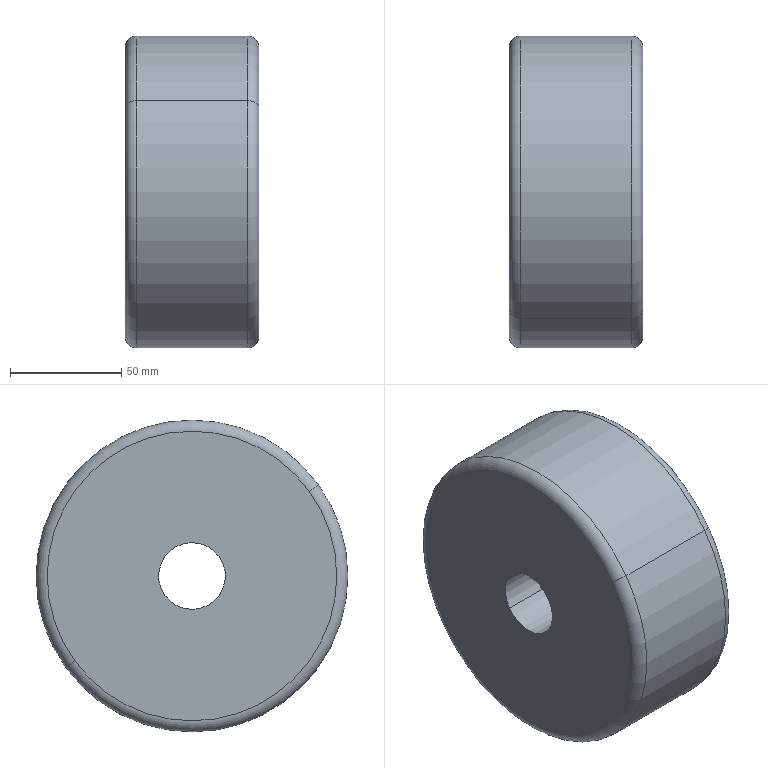Component | SolidWorks | TrashCanWheel-3 | 1 solid | 10 faces | box 60 x 140 x 140 mm | volume 876573 mm3 | torus 4 | cylinder 4 | plane 2 | commonest cylinder face diameters 30 x2 140 x2
build123d program:
from build123d import *

# Parameters (mm, degrees)
SKETCH1_R           = 70
SKETCH1_R_2         = 15
BOSS_EXTRUDE1_DEPTH = 60
FILLET1_R           = 5


with BuildPart() as part:
    # Sketch1 → Boss-Extrude1 (new body)
    with BuildSketch(Plane.XY):
        Circle(SKETCH1_R)
        Circle(SKETCH1_R_2, mode=Mode.SUBTRACT)
    extrude(amount=BOSS_EXTRUDE1_DEPTH)

    # Fillet1
    fillet1_edges = [part.edges().sort_by_distance(p)[0] for p in [
        (-70, 0, 0),
        (-70, 0, 60),
    ]]
    fillet(fillet1_edges, radius=FILLET1_R)


solid = part.part

# Placed as in the assembly
solid = solid.moved(Location((-414.371, -1323.331, 8.161), (0, 90, 0)))
STEP:
#1=CARTESIAN_POINT('',(-16.117,-49.866,-1.293));
#2=VERTEX_POINT('',#1);
#3=CARTESIAN_POINT('',(-16.117,-54.333,1.935));
#4=VERTEX_POINT('',#3);
#5=CARTESIAN_POINT('',(-16.117,-52.1,0.3213));
#6=DIRECTION('',(1.,0.,-0.));
#7=DIRECTION('',(0.,-0.8105,0.5857));
#8=AXIS2_PLACEMENT_3D('',#5,#6,#7);
#9=CIRCLE('',#8,2.756);
#10=EDGE_CURVE('',#2,#4,#9,.T.);
#11=ORIENTED_EDGE('',*,*,#10,.F.);
#12=CARTESIAN_POINT('',(-16.314,-50.025,-1.177));
#13=VERTEX_POINT('',#12);
#14=CARTESIAN_POINT('',(-16.117,-50.025,-1.177));
#15=DIRECTION('',(0.,0.5857,0.8105));
#16=DIRECTION('',(0.,-0.8105,0.5857));
#17=AXIS2_PLACEMENT_3D('',#14,#15,#16);
#18=CIRCLE('',#17,0.1969);
#19=EDGE_CURVE('',#2,#13,#18,.T.);
#20=ORIENTED_EDGE('',*,*,#19,.T.);
#21=CARTESIAN_POINT('',(-16.314,-54.174,1.82));
#22=VERTEX_POINT('',#21);
#23=CARTESIAN_POINT('',(-16.314,-52.1,0.3213));
#24=DIRECTION('',(-1.,-0.,0.));
#25=DIRECTION('',(0.,-0.8105,0.5857));
#26=AXIS2_PLACEMENT_3D('',#23,#24,#25);
#27=CIRCLE('',#26,2.559);
#28=EDGE_CURVE('',#22,#13,#27,.T.);
#29=ORIENTED_EDGE('',*,*,#28,.F.);
#30=CARTESIAN_POINT('',(-16.117,-54.174,1.82));
#31=DIRECTION('',(-0.,-0.5857,-0.8105));
#32=DIRECTION('',(0.,0.8105,-0.5857));
#33=AXIS2_PLACEMENT_3D('',#30,#31,#32);
#34=CIRCLE('',#33,0.1969);
#35=EDGE_CURVE('',#4,#22,#34,.T.);
#36=ORIENTED_EDGE('',*,*,#35,.F.);
#37=EDGE_LOOP('',(#11,#20,#29,#36));
#38=FACE_OUTER_BOUND('',#37,.T.);
#39=CARTESIAN_POINT('',(-16.117,-52.1,0.3213));
#40=DIRECTION('',(-1.,-0.,0.));
#41=DIRECTION('',(0.,-0.8105,0.5857));
#42=AXIS2_PLACEMENT_3D('',#39,#40,#41);
#43=TOROIDAL_SURFACE('',#42,2.559,0.1969);
#44=ADVANCED_FACE('',(#38),#43,.T.);
#45=CARTESIAN_POINT('',(-13.952,-50.025,-1.177));
#46=VERTEX_POINT('',#45);
#47=CARTESIAN_POINT('',(-13.952,-54.174,1.82));
#48=VERTEX_POINT('',#47);
#49=CARTESIAN_POINT('',(-13.952,-52.1,0.3213));
#50=DIRECTION('',(1.,0.,-0.));
#51=DIRECTION('',(0.,-0.8105,0.5857));
#52=AXIS2_PLACEMENT_3D('',#49,#50,#51);
#53=CIRCLE('',#52,2.559);
#54=EDGE_CURVE('',#46,#48,#53,.T.);
#55=ORIENTED_EDGE('',*,*,#54,.F.);
#56=CARTESIAN_POINT('',(-14.148,-49.866,-1.293));
#57=VERTEX_POINT('',#56);
#58=CARTESIAN_POINT('',(-14.148,-50.025,-1.177));
#59=DIRECTION('',(0.,0.5857,0.8105));
#60=DIRECTION('',(0.,-0.8105,0.5857));
#61=AXIS2_PLACEMENT_3D('',#58,#59,#60);
#62=CIRCLE('',#61,0.1969);
#63=EDGE_CURVE('',#46,#57,#62,.T.);
#64=ORIENTED_EDGE('',*,*,#63,.T.);
#65=CARTESIAN_POINT('',(-14.148,-54.333,1.935));
#66=VERTEX_POINT('',#65);
#67=CARTESIAN_POINT('',(-14.148,-52.1,0.3213));
#68=DIRECTION('',(-1.,-0.,0.));
#69=DIRECTION('',(0.,-0.8105,0.5857));
#70=AXIS2_PLACEMENT_3D('',#67,#68,#69);
#71=CIRCLE('',#70,2.756);
#72=EDGE_CURVE('',#66,#57,#71,.T.);
#73=ORIENTED_EDGE('',*,*,#72,.F.);
#74=CARTESIAN_POINT('',(-14.148,-54.174,1.82));
#75=DIRECTION('',(-0.,-0.5857,-0.8105));
#76=DIRECTION('',(0.,0.8105,-0.5857));
#77=AXIS2_PLACEMENT_3D('',#74,#75,#76);
#78=CIRCLE('',#77,0.1969);
#79=EDGE_CURVE('',#48,#66,#78,.T.);
#80=ORIENTED_EDGE('',*,*,#79,.F.);
#81=EDGE_LOOP('',(#55,#64,#73,#80));
#82=FACE_OUTER_BOUND('',#81,.T.);
#83=CARTESIAN_POINT('',(-14.148,-52.1,0.3213));
#84=DIRECTION('',(-1.,-0.,0.));
#85=DIRECTION('',(0.,-0.8105,0.5857));
#86=AXIS2_PLACEMENT_3D('',#83,#84,#85);
#87=TOROIDAL_SURFACE('',#86,2.559,0.1969);
#88=ADVANCED_FACE('',(#82),#87,.T.);
#89=CARTESIAN_POINT('',(-16.314,-51.621,-0.02458));
#90=VERTEX_POINT('',#89);
#91=CARTESIAN_POINT('',(-16.314,-52.578,0.6672));
#92=VERTEX_POINT('',#91);
#93=CARTESIAN_POINT('',(-16.314,-52.1,0.3213));
#94=DIRECTION('',(-1.,-0.,0.));
#95=DIRECTION('',(0.,-0.8105,0.5857));
#96=AXIS2_PLACEMENT_3D('',#93,#94,#95);
#97=CIRCLE('',#96,0.5906);
#98=EDGE_CURVE('',#90,#92,#97,.T.);
#99=ORIENTED_EDGE('',*,*,#98,.T.);
#100=CARTESIAN_POINT('',(-13.952,-52.578,0.6672));
#101=VERTEX_POINT('',#100);
#102=CARTESIAN_POINT('',(-16.314,-52.578,0.6672));
#103=DIRECTION('',(1.,0.,-0.));
#104=VECTOR('',#103,39.37);
#105=LINE('',#102,#104);
#106=EDGE_CURVE('',#92,#101,#105,.T.);
#107=ORIENTED_EDGE('',*,*,#106,.T.);
#108=CARTESIAN_POINT('',(-13.952,-51.621,-0.02458));
#109=VERTEX_POINT('',#108);
#110=CARTESIAN_POINT('',(-13.952,-52.1,0.3213));
#111=DIRECTION('',(-1.,-0.,0.));
#112=DIRECTION('',(0.,-0.8105,0.5857));
#113=AXIS2_PLACEMENT_3D('',#110,#111,#112);
#114=CIRCLE('',#113,0.5906);
#115=EDGE_CURVE('',#109,#101,#114,.T.);
#116=ORIENTED_EDGE('',*,*,#115,.F.);
#117=CARTESIAN_POINT('',(-16.314,-51.621,-0.02458));
#118=DIRECTION('',(1.,0.,-0.));
#119=VECTOR('',#118,39.37);
#120=LINE('',#117,#119);
#121=EDGE_CURVE('',#90,#109,#120,.T.);
#122=ORIENTED_EDGE('',*,*,#121,.F.);
#123=EDGE_LOOP('',(#99,#107,#116,#122));
#124=FACE_OUTER_BOUND('',#123,.T.);
#125=CARTESIAN_POINT('',(-16.314,-52.1,0.3213));
#126=DIRECTION('',(1.,0.,-0.));
#127=DIRECTION('',(0.,0.8105,-0.5857));
#128=AXIS2_PLACEMENT_3D('',#125,#126,#127);
#129=CYLINDRICAL_SURFACE('',#128,0.5906);
#130=ADVANCED_FACE('',(#124),#129,.F.);
#131=ORIENTED_EDGE('',*,*,#10,.T.);
#132=CARTESIAN_POINT('',(-16.314,-54.333,1.935));
#133=DIRECTION('',(1.,0.,-0.));
#134=VECTOR('',#133,39.37);
#135=LINE('',#132,#134);
#136=EDGE_CURVE('',#4,#66,#135,.T.);
#137=ORIENTED_EDGE('',*,*,#136,.T.);
#138=ORIENTED_EDGE('',*,*,#72,.T.);
#139=CARTESIAN_POINT('',(-16.314,-49.866,-1.293));
#140=DIRECTION('',(1.,0.,-0.));
#141=VECTOR('',#140,39.37);
#142=LINE('',#139,#141);
#143=EDGE_CURVE('',#2,#57,#142,.T.);
#144=ORIENTED_EDGE('',*,*,#143,.F.);
#145=EDGE_LOOP('',(#131,#137,#138,#144));
#146=FACE_OUTER_BOUND('',#145,.T.);
#147=CARTESIAN_POINT('',(-16.314,-52.1,0.3213));
#148=DIRECTION('',(1.,0.,-0.));
#149=DIRECTION('',(0.,0.8105,-0.5857));
#150=AXIS2_PLACEMENT_3D('',#147,#148,#149);
#151=CYLINDRICAL_SURFACE('',#150,2.756);
#152=ADVANCED_FACE('',(#146),#151,.T.);
#153=ORIENTED_EDGE('',*,*,#28,.T.);
#154=CARTESIAN_POINT('',(-16.314,-52.1,0.3213));
#155=DIRECTION('',(-1.,-0.,0.));
#156=DIRECTION('',(0.,-0.8105,0.5857));
#157=AXIS2_PLACEMENT_3D('',#154,#155,#156);
#158=CIRCLE('',#157,2.559);
#159=EDGE_CURVE('',#13,#22,#158,.T.);
#160=ORIENTED_EDGE('',*,*,#159,.T.);
#161=EDGE_LOOP('',(#153,#160));
#162=FACE_OUTER_BOUND('',#161,.T.);
#163=ORIENTED_EDGE('',*,*,#98,.F.);
#164=CARTESIAN_POINT('',(-16.314,-52.1,0.3213));
#165=DIRECTION('',(-1.,-0.,0.));
#166=DIRECTION('',(0.,-0.8105,0.5857));
#167=AXIS2_PLACEMENT_3D('',#164,#165,#166);
#168=CIRCLE('',#167,0.5906);
#169=EDGE_CURVE('',#92,#90,#168,.T.);
#170=ORIENTED_EDGE('',*,*,#169,.F.);
#171=EDGE_LOOP('',(#163,#170));
#172=FACE_BOUND('',#171,.T.);
#173=CARTESIAN_POINT('',(-16.314,-52.1,0.3213));
#174=DIRECTION('',(-1.,-0.,0.));
#175=DIRECTION('',(0.,-0.8105,0.5857));
#176=AXIS2_PLACEMENT_3D('',#173,#174,#175);
#177=PLANE('',#176);
#178=ADVANCED_FACE('',(#162,#172),#177,.T.);
#179=CARTESIAN_POINT('',(-13.952,-52.1,0.3213));
#180=DIRECTION('',(1.,0.,-0.));
#181=DIRECTION('',(0.,-0.8105,0.5857));
#182=AXIS2_PLACEMENT_3D('',#179,#180,#181);
#183=CIRCLE('',#182,2.559);
#184=EDGE_CURVE('',#48,#46,#183,.T.);
#185=ORIENTED_EDGE('',*,*,#184,.T.);
#186=ORIENTED_EDGE('',*,*,#54,.T.);
#187=EDGE_LOOP('',(#185,#186));
#188=FACE_OUTER_BOUND('',#187,.T.);
#189=ORIENTED_EDGE('',*,*,#115,.T.);
#190=CARTESIAN_POINT('',(-13.952,-52.1,0.3213));
#191=DIRECTION('',(-1.,-0.,0.));
#192=DIRECTION('',(0.,-0.8105,0.5857));
#193=AXIS2_PLACEMENT_3D('',#190,#191,#192);
#194=CIRCLE('',#193,0.5906);
#195=EDGE_CURVE('',#101,#109,#194,.T.);
#196=ORIENTED_EDGE('',*,*,#195,.T.);
#197=EDGE_LOOP('',(#189,#196));
#198=FACE_BOUND('',#197,.T.);
#199=CARTESIAN_POINT('',(-13.952,-52.1,0.3213));
#200=DIRECTION('',(-1.,-0.,0.));
#201=DIRECTION('',(0.,-0.8105,0.5857));
#202=AXIS2_PLACEMENT_3D('',#199,#200,#201);
#203=PLANE('',#202);
#204=ADVANCED_FACE('',(#188,#198),#203,.F.);
#205=ORIENTED_EDGE('',*,*,#136,.F.);
#206=CARTESIAN_POINT('',(-16.117,-52.1,0.3213));
#207=DIRECTION('',(1.,0.,-0.));
#208=DIRECTION('',(0.,-0.8105,0.5857));
#209=AXIS2_PLACEMENT_3D('',#206,#207,#208);
#210=CIRCLE('',#209,2.756);
#211=EDGE_CURVE('',#4,#2,#210,.T.);
#212=ORIENTED_EDGE('',*,*,#211,.T.);
#213=ORIENTED_EDGE('',*,*,#143,.T.);
#214=CARTESIAN_POINT('',(-14.148,-52.1,0.3213));
#215=DIRECTION('',(-1.,-0.,0.));
#216=DIRECTION('',(0.,-0.8105,0.5857));
#217=AXIS2_PLACEMENT_3D('',#214,#215,#216);
#218=CIRCLE('',#217,2.756);
#219=EDGE_CURVE('',#57,#66,#218,.T.);
#220=ORIENTED_EDGE('',*,*,#219,.T.);
#221=EDGE_LOOP('',(#205,#212,#213,#220));
#222=FACE_OUTER_BOUND('',#221,.T.);
#223=CARTESIAN_POINT('',(-16.314,-52.1,0.3213));
#224=DIRECTION('',(1.,0.,-0.));
#225=DIRECTION('',(0.,0.8105,-0.5857));
#226=AXIS2_PLACEMENT_3D('',#223,#224,#225);
#227=CYLINDRICAL_SURFACE('',#226,2.756);
#228=ADVANCED_FACE('',(#222),#227,.T.);
#229=ORIENTED_EDGE('',*,*,#106,.F.);
#230=ORIENTED_EDGE('',*,*,#169,.T.);
#231=ORIENTED_EDGE('',*,*,#121,.T.);
#232=ORIENTED_EDGE('',*,*,#195,.F.);
#233=EDGE_LOOP('',(#229,#230,#231,#232));
#234=FACE_OUTER_BOUND('',#233,.T.);
#235=CARTESIAN_POINT('',(-16.314,-52.1,0.3213));
#236=DIRECTION('',(1.,0.,-0.));
#237=DIRECTION('',(0.,0.8105,-0.5857));
#238=AXIS2_PLACEMENT_3D('',#235,#236,#237);
#239=CYLINDRICAL_SURFACE('',#238,0.5906);
#240=ADVANCED_FACE('',(#234),#239,.F.);
#241=ORIENTED_EDGE('',*,*,#63,.F.);
#242=ORIENTED_EDGE('',*,*,#184,.F.);
#243=ORIENTED_EDGE('',*,*,#79,.T.);
#244=ORIENTED_EDGE('',*,*,#219,.F.);
#245=EDGE_LOOP('',(#241,#242,#243,#244));
#246=FACE_OUTER_BOUND('',#245,.T.);
#247=CARTESIAN_POINT('',(-14.148,-52.1,0.3213));
#248=DIRECTION('',(-1.,-0.,0.));
#249=DIRECTION('',(0.,-0.8105,0.5857));
#250=AXIS2_PLACEMENT_3D('',#247,#248,#249);
#251=TOROIDAL_SURFACE('',#250,2.559,0.1969);
#252=ADVANCED_FACE('',(#246),#251,.T.);
#253=ORIENTED_EDGE('',*,*,#19,.F.);
#254=ORIENTED_EDGE('',*,*,#211,.F.);
#255=ORIENTED_EDGE('',*,*,#35,.T.);
#256=ORIENTED_EDGE('',*,*,#159,.F.);
#257=EDGE_LOOP('',(#253,#254,#255,#256));
#258=FACE_OUTER_BOUND('',#257,.T.);
#259=CARTESIAN_POINT('',(-16.117,-52.1,0.3213));
#260=DIRECTION('',(-1.,-0.,0.));
#261=DIRECTION('',(0.,-0.8105,0.5857));
#262=AXIS2_PLACEMENT_3D('',#259,#260,#261);
#263=TOROIDAL_SURFACE('',#262,2.559,0.1969);
#264=ADVANCED_FACE('',(#258),#263,.T.);
#265=CLOSED_SHELL('',(#44,#88,#130,#152,#178,#204,#228,#240,#252,#264));
#266=MANIFOLD_SOLID_BREP('',#265);
#267=CARTESIAN_POINT('',(0.,0.,0.));
#268=DIRECTION('',(0.,0.,1.));
#269=DIRECTION('',(1.,0.,0.));
#270=AXIS2_PLACEMENT_3D('',#267,#268,#269);
#271=(LENGTH_UNIT()NAMED_UNIT(*)SI_UNIT($,.METRE.));
#272=LENGTH_MEASURE_WITH_UNIT(LENGTH_MEASURE(0.0254),#271);
#273=DIMENSIONAL_EXPONENTS(1.,0.,0.,0.,0.,0.,0.);
#274=(CONVERSION_BASED_UNIT('',#272)LENGTH_UNIT()NAMED_UNIT(#273));
#275=UNCERTAINTY_MEASURE_WITH_UNIT(LENGTH_MEASURE(0.00001),#274,'','');
#276=(NAMED_UNIT(*)PLANE_ANGLE_UNIT()SI_UNIT($,.RADIAN.));
#277=(NAMED_UNIT(*)SI_UNIT($,.STERADIAN.)SOLID_ANGLE_UNIT());
#278=(GEOMETRIC_REPRESENTATION_CONTEXT(3)GLOBAL_UNCERTAINTY_ASSIGNED_CONTEXT((#275))GLOBAL_UNIT_ASSIGNED_CONTEXT((#274,#276,#277))REPRESENTATION_CONTEXT('',''));
#279=ADVANCED_BREP_SHAPE_REPRESENTATION('',(#266,#270),#278);
#280=COLOUR_RGB('',0.7922,0.8196,0.9333);
#281=FILL_AREA_STYLE_COLOUR('',#280);
#282=FILL_AREA_STYLE('',(#281));
#283=SURFACE_STYLE_FILL_AREA(#282);
#284=SURFACE_SIDE_STYLE('',(#283));
#285=SURFACE_STYLE_USAGE(.BOTH.,#284);
#286=PRESENTATION_STYLE_ASSIGNMENT((#285));
#287=STYLED_ITEM('',(#286),#266);
#288=(LENGTH_UNIT()NAMED_UNIT(*)SI_UNIT($,.METRE.));
#289=LENGTH_MEASURE_WITH_UNIT(LENGTH_MEASURE(0.0254),#288);
#290=DIMENSIONAL_EXPONENTS(1.,0.,0.,0.,0.,0.,0.);
#291=(CONVERSION_BASED_UNIT('',#289)LENGTH_UNIT()NAMED_UNIT(#290));
#292=UNCERTAINTY_MEASURE_WITH_UNIT(LENGTH_MEASURE(0.00001),#291,'','');
#293=(NAMED_UNIT(*)PLANE_ANGLE_UNIT()SI_UNIT($,.RADIAN.));
#294=(NAMED_UNIT(*)SI_UNIT($,.STERADIAN.)SOLID_ANGLE_UNIT());
#295=(GEOMETRIC_REPRESENTATION_CONTEXT(3)GLOBAL_UNCERTAINTY_ASSIGNED_CONTEXT((#292))GLOBAL_UNIT_ASSIGNED_CONTEXT((#291,#293,#294))REPRESENTATION_CONTEXT('',''));
#296=MECHANICAL_DESIGN_GEOMETRIC_PRESENTATION_REPRESENTATION('',(#287),#295);
#297=PRESENTATION_LAYER_ASSIGNMENT('','',(#287));